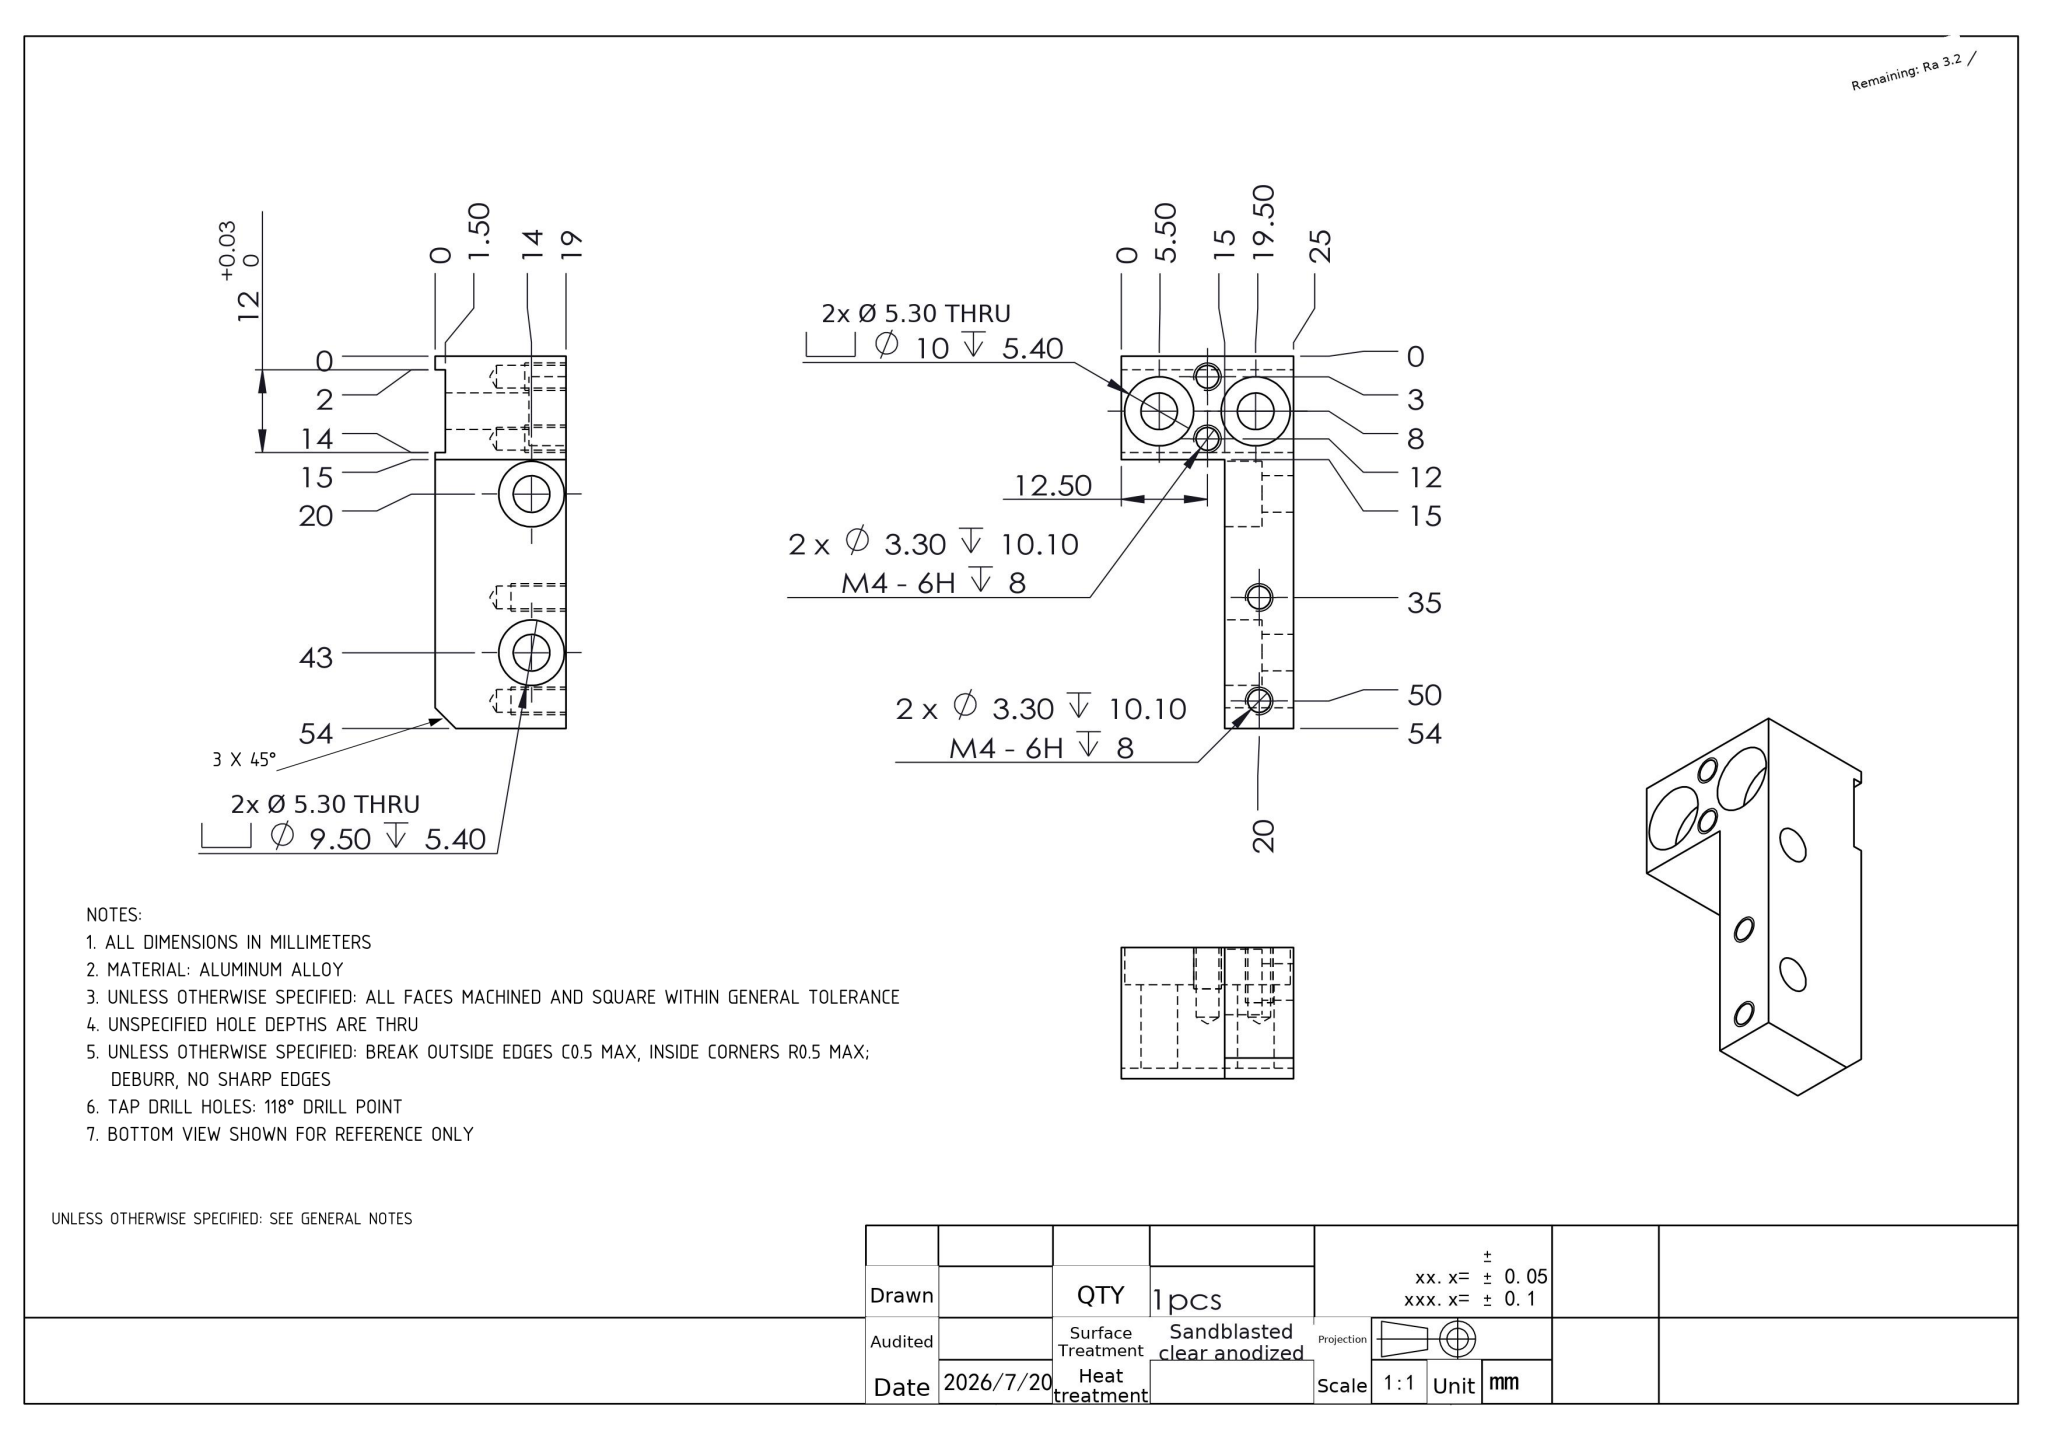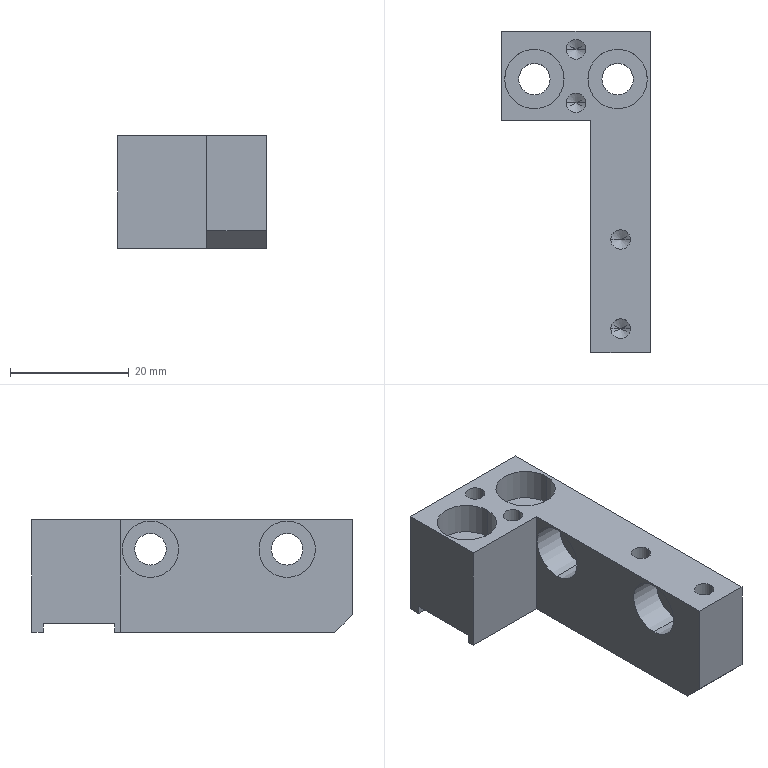Part | NX | mm | 1 solid | 49 faces | box 25 x 54 x 19 mm | volume 11333 mm3 | cylinder 24 | plane 17 | cone 8 | commonest cylinder face diameters 3.3 x8 5.3 x8 9.5 x4 10 x4